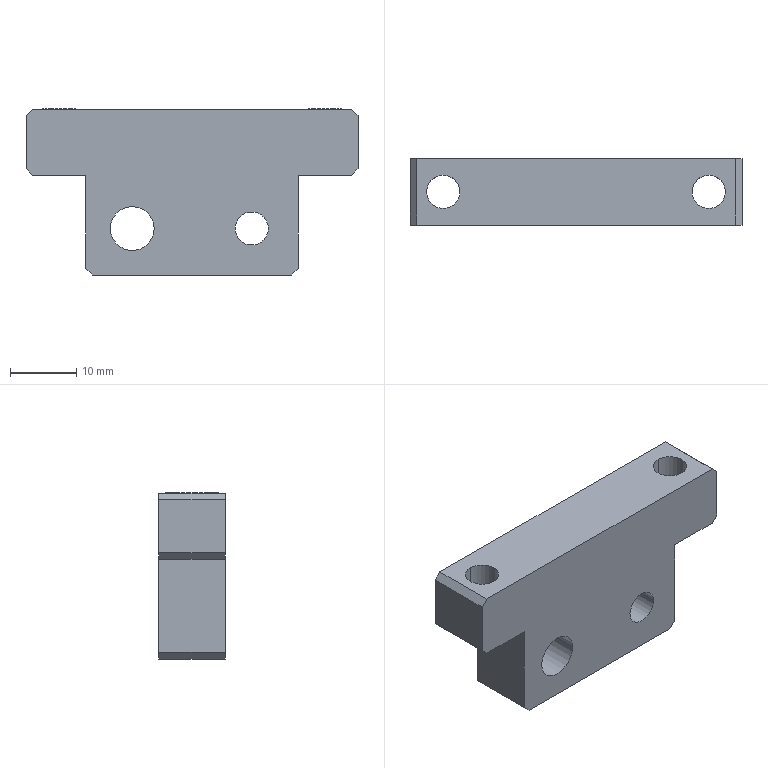Component | SolidWorks | 8TC-A17001-90-08AdjustmentSeat-1 | 1 solid | 24 faces | box 50 x 10 x 25 mm | volume 8839 mm3 | plane 16 | cylinder 8 | commonest cylinder face diameters 5 x6 6.6 x2 | material A3
build123d program:
from build123d import *

# Parameters (mm, degrees)
BOSS_EXTRUDE1_DEPTH                        = 5
THREADED_HOLE_DRILL_FOR_M6_THREADED_HOLE_D = 5
M6_TAPPED_HOLE1_D                          = 5
M6_CLEARANCE_HOLE_1_D                      = 6.6
CHAMFER1_SIZE                              = 1


with BuildPart() as part:
    # Sketch1 → Boss-Extrude1 (new, symmetric)
    with BuildSketch(Plane.XY):
        Polygon((-25, 10), (-16, 10), (-16, 25), (16, 25), (16, 10), (25, 10), (25, 0), (-25, 0), align=None)
    extrude(amount=BOSS_EXTRUDE1_DEPTH, both=True)

    # Threaded Hole Drill for M6 Threaded Hole (through all)
    with Locations(Plane(origin=(0, 10, 0), x_dir=(1, 0, 0), z_dir=(0, 1, 0))):
        with Locations((-20, 0), (20, 0)):
            Hole(THREADED_HOLE_DRILL_FOR_M6_THREADED_HOLE_D / 2)

    # M6 Tapped Hole1 (through all)
    with Locations(Plane.XY.offset(5)):
        with Locations((9, 18)):
            Hole(M6_TAPPED_HOLE1_D / 2)

    # M6 Clearance Hole 1 (through all)
    with Locations(Plane.XY.offset(5)):
        with Locations((-9, 18)):
            Hole(M6_CLEARANCE_HOLE_1_D / 2)

    # Chamfer1
    chamfer1_edges = [part.edges().sort_by_distance(p)[0] for p in [
        (-25, 10, 0),
        (-16, 25, 0),
        (16, 25, 0),
        (25, 10, 0),
        (25, 0, 0),
        (-25, 0, 0),
    ]]
    chamfer(chamfer1_edges, length=CHAMFER1_SIZE)


solid = part.part

# Placed as in the assembly
solid = solid.moved(Location((0, 100, 0), (-90, 0, 0)))
STEP:
#1=COLOUR_RGB('',0.7922,0.8196,0.9333);
#2=FILL_AREA_STYLE_COLOUR('',#1);
#3=FILL_AREA_STYLE('',(#2));
#4=SURFACE_STYLE_FILL_AREA(#3);
#5=SURFACE_SIDE_STYLE('',(#4));
#6=SURFACE_STYLE_USAGE(.BOTH.,#5);
#7=PRESENTATION_STYLE_ASSIGNMENT((#6));
#8=CARTESIAN_POINT('',(-0.4843,3.74,-0.7087));
#9=VERTEX_POINT('',#8);
#10=CARTESIAN_POINT('',(-0.2244,3.74,-0.7087));
#11=VERTEX_POINT('',#10);
#12=CARTESIAN_POINT('',(-0.3543,3.74,-0.7087));
#13=DIRECTION('',(0.,1.,-0.));
#14=DIRECTION('',(1.,0.,0.));
#15=AXIS2_PLACEMENT_3D('',#12,#13,#14);
#16=CIRCLE('',#15,0.1299);
#17=EDGE_CURVE('',#9,#11,#16,.T.);
#18=ORIENTED_EDGE('',*,*,#17,.F.);
#19=CARTESIAN_POINT('',(-0.4843,4.134,-0.7087));
#20=VERTEX_POINT('',#19);
#21=CARTESIAN_POINT('',(-0.4843,4.134,-0.7087));
#22=DIRECTION('',(0.,1.,-0.));
#23=VECTOR('',#22,39.37);
#24=LINE('',#21,#23);
#25=EDGE_CURVE('',#9,#20,#24,.T.);
#26=ORIENTED_EDGE('',*,*,#25,.T.);
#27=CARTESIAN_POINT('',(-0.2244,4.134,-0.7087));
#28=VERTEX_POINT('',#27);
#29=CARTESIAN_POINT('',(-0.3543,4.134,-0.7087));
#30=DIRECTION('',(0.,1.,-0.));
#31=DIRECTION('',(1.,0.,0.));
#32=AXIS2_PLACEMENT_3D('',#29,#30,#31);
#33=CIRCLE('',#32,0.1299);
#34=EDGE_CURVE('',#20,#28,#33,.T.);
#35=ORIENTED_EDGE('',*,*,#34,.T.);
#36=CARTESIAN_POINT('',(-0.2244,4.134,-0.7087));
#37=DIRECTION('',(0.,1.,-0.));
#38=VECTOR('',#37,39.37);
#39=LINE('',#36,#38);
#40=EDGE_CURVE('',#11,#28,#39,.T.);
#41=ORIENTED_EDGE('',*,*,#40,.F.);
#42=EDGE_LOOP('',(#18,#26,#35,#41));
#43=FACE_OUTER_BOUND('',#42,.T.);
#44=CARTESIAN_POINT('',(-0.3543,4.134,-0.7087));
#45=DIRECTION('',(0.,1.,-0.));
#46=DIRECTION('',(1.,0.,0.));
#47=AXIS2_PLACEMENT_3D('',#44,#45,#46);
#48=CYLINDRICAL_SURFACE('',#47,0.1299);
#49=ADVANCED_FACE('',(#43),#48,.F.);
#50=CARTESIAN_POINT('',(0.2559,3.74,-0.7087));
#51=VERTEX_POINT('',#50);
#52=CARTESIAN_POINT('',(0.4528,3.74,-0.7087));
#53=VERTEX_POINT('',#52);
#54=CARTESIAN_POINT('',(0.3543,3.74,-0.7087));
#55=DIRECTION('',(0.,1.,-0.));
#56=DIRECTION('',(1.,0.,0.));
#57=AXIS2_PLACEMENT_3D('',#54,#55,#56);
#58=CIRCLE('',#57,0.09843);
#59=EDGE_CURVE('',#51,#53,#58,.T.);
#60=ORIENTED_EDGE('',*,*,#59,.F.);
#61=CARTESIAN_POINT('',(0.2559,4.134,-0.7087));
#62=VERTEX_POINT('',#61);
#63=CARTESIAN_POINT('',(0.2559,4.134,-0.7087));
#64=DIRECTION('',(0.,1.,-0.));
#65=VECTOR('',#64,39.37);
#66=LINE('',#63,#65);
#67=EDGE_CURVE('',#51,#62,#66,.T.);
#68=ORIENTED_EDGE('',*,*,#67,.T.);
#69=CARTESIAN_POINT('',(0.4528,4.134,-0.7087));
#70=VERTEX_POINT('',#69);
#71=CARTESIAN_POINT('',(0.3543,4.134,-0.7087));
#72=DIRECTION('',(0.,1.,-0.));
#73=DIRECTION('',(1.,0.,0.));
#74=AXIS2_PLACEMENT_3D('',#71,#72,#73);
#75=CIRCLE('',#74,0.09843);
#76=EDGE_CURVE('',#62,#70,#75,.T.);
#77=ORIENTED_EDGE('',*,*,#76,.T.);
#78=CARTESIAN_POINT('',(0.4528,4.134,-0.7087));
#79=DIRECTION('',(0.,1.,-0.));
#80=VECTOR('',#79,39.37);
#81=LINE('',#78,#80);
#82=EDGE_CURVE('',#53,#70,#81,.T.);
#83=ORIENTED_EDGE('',*,*,#82,.F.);
#84=EDGE_LOOP('',(#60,#68,#77,#83));
#85=FACE_OUTER_BOUND('',#84,.T.);
#86=CARTESIAN_POINT('',(0.3543,4.134,-0.7087));
#87=DIRECTION('',(0.,1.,-0.));
#88=DIRECTION('',(1.,0.,0.));
#89=AXIS2_PLACEMENT_3D('',#86,#87,#88);
#90=CYLINDRICAL_SURFACE('',#89,0.09843);
#91=ADVANCED_FACE('',(#85),#90,.F.);
#92=CARTESIAN_POINT('',(-0.7874,3.839,0.));
#93=VERTEX_POINT('',#92);
#94=CARTESIAN_POINT('',(-0.7874,4.035,0.));
#95=VERTEX_POINT('',#94);
#96=CARTESIAN_POINT('',(-0.7874,3.937,0.));
#97=DIRECTION('',(0.,0.,-1.));
#98=DIRECTION('',(0.,1.,0.));
#99=AXIS2_PLACEMENT_3D('',#96,#97,#98);
#100=CIRCLE('',#99,0.09843);
#101=EDGE_CURVE('',#93,#95,#100,.T.);
#102=ORIENTED_EDGE('',*,*,#101,.F.);
#103=CARTESIAN_POINT('',(-0.7874,3.839,-0.3937));
#104=VERTEX_POINT('',#103);
#105=CARTESIAN_POINT('',(-0.7874,3.839,-0.3937));
#106=DIRECTION('',(0.,0.,-1.));
#107=VECTOR('',#106,39.37);
#108=LINE('',#105,#107);
#109=EDGE_CURVE('',#93,#104,#108,.T.);
#110=ORIENTED_EDGE('',*,*,#109,.T.);
#111=CARTESIAN_POINT('',(-0.7874,4.035,-0.3937));
#112=VERTEX_POINT('',#111);
#113=CARTESIAN_POINT('',(-0.7874,3.937,-0.3937));
#114=DIRECTION('',(0.,0.,-1.));
#115=DIRECTION('',(0.,1.,0.));
#116=AXIS2_PLACEMENT_3D('',#113,#114,#115);
#117=CIRCLE('',#116,0.09843);
#118=EDGE_CURVE('',#104,#112,#117,.T.);
#119=ORIENTED_EDGE('',*,*,#118,.T.);
#120=CARTESIAN_POINT('',(-0.7874,4.035,-0.3937));
#121=DIRECTION('',(0.,0.,-1.));
#122=VECTOR('',#121,39.37);
#123=LINE('',#120,#122);
#124=EDGE_CURVE('',#95,#112,#123,.T.);
#125=ORIENTED_EDGE('',*,*,#124,.F.);
#126=EDGE_LOOP('',(#102,#110,#119,#125));
#127=FACE_OUTER_BOUND('',#126,.T.);
#128=CARTESIAN_POINT('',(-0.7874,3.937,-0.3937));
#129=DIRECTION('',(0.,0.,-1.));
#130=DIRECTION('',(0.,1.,0.));
#131=AXIS2_PLACEMENT_3D('',#128,#129,#130);
#132=CYLINDRICAL_SURFACE('',#131,0.09843);
#133=ADVANCED_FACE('',(#127),#132,.F.);
#134=CARTESIAN_POINT('',(0.7874,3.839,0.));
#135=VERTEX_POINT('',#134);
#136=CARTESIAN_POINT('',(0.7874,4.035,0.));
#137=VERTEX_POINT('',#136);
#138=CARTESIAN_POINT('',(0.7874,3.937,0.));
#139=DIRECTION('',(0.,0.,-1.));
#140=DIRECTION('',(0.,1.,0.));
#141=AXIS2_PLACEMENT_3D('',#138,#139,#140);
#142=CIRCLE('',#141,0.09843);
#143=EDGE_CURVE('',#135,#137,#142,.T.);
#144=ORIENTED_EDGE('',*,*,#143,.F.);
#145=CARTESIAN_POINT('',(0.7874,3.839,-0.3937));
#146=VERTEX_POINT('',#145);
#147=CARTESIAN_POINT('',(0.7874,3.839,-0.3937));
#148=DIRECTION('',(0.,0.,-1.));
#149=VECTOR('',#148,39.37);
#150=LINE('',#147,#149);
#151=EDGE_CURVE('',#135,#146,#150,.T.);
#152=ORIENTED_EDGE('',*,*,#151,.T.);
#153=CARTESIAN_POINT('',(0.7874,4.035,-0.3937));
#154=VERTEX_POINT('',#153);
#155=CARTESIAN_POINT('',(0.7874,3.937,-0.3937));
#156=DIRECTION('',(0.,0.,-1.));
#157=DIRECTION('',(0.,1.,0.));
#158=AXIS2_PLACEMENT_3D('',#155,#156,#157);
#159=CIRCLE('',#158,0.09843);
#160=EDGE_CURVE('',#146,#154,#159,.T.);
#161=ORIENTED_EDGE('',*,*,#160,.T.);
#162=CARTESIAN_POINT('',(0.7874,4.035,-0.3937));
#163=DIRECTION('',(0.,0.,-1.));
#164=VECTOR('',#163,39.37);
#165=LINE('',#162,#164);
#166=EDGE_CURVE('',#137,#154,#165,.T.);
#167=ORIENTED_EDGE('',*,*,#166,.F.);
#168=EDGE_LOOP('',(#144,#152,#161,#167));
#169=FACE_OUTER_BOUND('',#168,.T.);
#170=CARTESIAN_POINT('',(0.7874,3.937,-0.3937));
#171=DIRECTION('',(0.,0.,-1.));
#172=DIRECTION('',(0.,1.,0.));
#173=AXIS2_PLACEMENT_3D('',#170,#171,#172);
#174=CYLINDRICAL_SURFACE('',#173,0.09843);
#175=ADVANCED_FACE('',(#169),#174,.F.);
#176=CARTESIAN_POINT('',(-0.9843,4.134,-0.3543));
#177=VERTEX_POINT('',#176);
#178=CARTESIAN_POINT('',(-0.9843,4.134,-0.03937));
#179=VERTEX_POINT('',#178);
#180=CARTESIAN_POINT('',(-0.9843,4.134,-0.3937));
#181=DIRECTION('',(-0.,0.,1.));
#182=VECTOR('',#181,39.37);
#183=LINE('',#180,#182);
#184=EDGE_CURVE('',#177,#179,#183,.T.);
#185=ORIENTED_EDGE('',*,*,#184,.F.);
#186=CARTESIAN_POINT('',(-0.9843,3.74,-0.3543));
#187=VERTEX_POINT('',#186);
#188=CARTESIAN_POINT('',(-0.9843,4.134,-0.3543));
#189=DIRECTION('',(-0.,-1.,0.));
#190=VECTOR('',#189,39.37);
#191=LINE('',#188,#190);
#192=EDGE_CURVE('',#177,#187,#191,.T.);
#193=ORIENTED_EDGE('',*,*,#192,.T.);
#194=CARTESIAN_POINT('',(-0.9843,3.74,-0.03937));
#195=VERTEX_POINT('',#194);
#196=CARTESIAN_POINT('',(-0.9843,3.74,-0.3937));
#197=DIRECTION('',(-0.,0.,1.));
#198=VECTOR('',#197,39.37);
#199=LINE('',#196,#198);
#200=EDGE_CURVE('',#187,#195,#199,.T.);
#201=ORIENTED_EDGE('',*,*,#200,.T.);
#202=CARTESIAN_POINT('',(-0.9843,4.134,-0.03937));
#203=DIRECTION('',(0.,1.,-0.));
#204=VECTOR('',#203,39.37);
#205=LINE('',#202,#204);
#206=EDGE_CURVE('',#195,#179,#205,.T.);
#207=ORIENTED_EDGE('',*,*,#206,.T.);
#208=EDGE_LOOP('',(#185,#193,#201,#207));
#209=FACE_OUTER_BOUND('',#208,.T.);
#210=CARTESIAN_POINT('',(-0.9843,4.134,-0.3937));
#211=DIRECTION('',(1.,-0.,0.));
#212=DIRECTION('',(-0.,-1.,0.));
#213=AXIS2_PLACEMENT_3D('',#210,#211,#212);
#214=PLANE('',#213);
#215=ADVANCED_FACE('',(#209),#214,.F.);
#216=CARTESIAN_POINT('',(-0.7874,3.937,0.));
#217=DIRECTION('',(0.,0.,-1.));
#218=DIRECTION('',(0.,1.,0.));
#219=AXIS2_PLACEMENT_3D('',#216,#217,#218);
#220=CIRCLE('',#219,0.09843);
#221=EDGE_CURVE('',#95,#93,#220,.T.);
#222=ORIENTED_EDGE('',*,*,#221,.T.);
#223=ORIENTED_EDGE('',*,*,#101,.T.);
#224=EDGE_LOOP('',(#222,#223));
#225=FACE_BOUND('',#224,.T.);
#226=CARTESIAN_POINT('',(0.7874,3.937,0.));
#227=DIRECTION('',(0.,0.,-1.));
#228=DIRECTION('',(0.,1.,0.));
#229=AXIS2_PLACEMENT_3D('',#226,#227,#228);
#230=CIRCLE('',#229,0.09843);
#231=EDGE_CURVE('',#137,#135,#230,.T.);
#232=ORIENTED_EDGE('',*,*,#231,.T.);
#233=ORIENTED_EDGE('',*,*,#143,.T.);
#234=EDGE_LOOP('',(#232,#233));
#235=FACE_BOUND('',#234,.T.);
#236=CARTESIAN_POINT('',(-0.9449,3.74,-0.));
#237=VERTEX_POINT('',#236);
#238=CARTESIAN_POINT('',(0.9449,3.74,0.));
#239=VERTEX_POINT('',#238);
#240=CARTESIAN_POINT('',(0.9843,3.74,0.));
#241=DIRECTION('',(1.,0.,0.));
#242=VECTOR('',#241,39.37);
#243=LINE('',#240,#242);
#244=EDGE_CURVE('',#237,#239,#243,.T.);
#245=ORIENTED_EDGE('',*,*,#244,.T.);
#246=CARTESIAN_POINT('',(0.9449,4.134,0.));
#247=VERTEX_POINT('',#246);
#248=CARTESIAN_POINT('',(0.9449,4.134,0.));
#249=DIRECTION('',(0.,1.,-0.));
#250=VECTOR('',#249,39.37);
#251=LINE('',#248,#250);
#252=EDGE_CURVE('',#239,#247,#251,.T.);
#253=ORIENTED_EDGE('',*,*,#252,.T.);
#254=CARTESIAN_POINT('',(-0.9449,4.134,-0.));
#255=VERTEX_POINT('',#254);
#256=CARTESIAN_POINT('',(0.9843,4.134,0.));
#257=DIRECTION('',(1.,0.,0.));
#258=VECTOR('',#257,39.37);
#259=LINE('',#256,#258);
#260=EDGE_CURVE('',#255,#247,#259,.T.);
#261=ORIENTED_EDGE('',*,*,#260,.F.);
#262=CARTESIAN_POINT('',(-0.9449,4.134,-0.));
#263=DIRECTION('',(-0.,-1.,0.));
#264=VECTOR('',#263,39.37);
#265=LINE('',#262,#264);
#266=EDGE_CURVE('',#255,#237,#265,.T.);
#267=ORIENTED_EDGE('',*,*,#266,.T.);
#268=EDGE_LOOP('',(#245,#253,#261,#267));
#269=FACE_OUTER_BOUND('',#268,.T.);
#270=CARTESIAN_POINT('',(0.9843,4.134,0.));
#271=DIRECTION('',(0.,-0.,-1.));
#272=DIRECTION('',(0.,1.,-0.));
#273=AXIS2_PLACEMENT_3D('',#270,#271,#272);
#274=PLANE('',#273);
#275=ADVANCED_FACE('',(#225,#235,#269),#274,.F.);
#276=CARTESIAN_POINT('',(0.9843,3.74,-0.03937));
#277=VERTEX_POINT('',#276);
#278=CARTESIAN_POINT('',(0.9843,3.74,-0.3543));
#279=VERTEX_POINT('',#278);
#280=CARTESIAN_POINT('',(0.9843,3.74,-0.3937));
#281=DIRECTION('',(0.,0.,-1.));
#282=VECTOR('',#281,39.37);
#283=LINE('',#280,#282);
#284=EDGE_CURVE('',#277,#279,#283,.T.);
#285=ORIENTED_EDGE('',*,*,#284,.T.);
#286=CARTESIAN_POINT('',(0.9843,4.134,-0.3543));
#287=VERTEX_POINT('',#286);
#288=CARTESIAN_POINT('',(0.9843,4.134,-0.3543));
#289=DIRECTION('',(0.,1.,-0.));
#290=VECTOR('',#289,39.37);
#291=LINE('',#288,#290);
#292=EDGE_CURVE('',#279,#287,#291,.T.);
#293=ORIENTED_EDGE('',*,*,#292,.T.);
#294=CARTESIAN_POINT('',(0.9843,4.134,-0.03937));
#295=VERTEX_POINT('',#294);
#296=CARTESIAN_POINT('',(0.9843,4.134,-0.3937));
#297=DIRECTION('',(0.,0.,-1.));
#298=VECTOR('',#297,39.37);
#299=LINE('',#296,#298);
#300=EDGE_CURVE('',#295,#287,#299,.T.);
#301=ORIENTED_EDGE('',*,*,#300,.F.);
#302=CARTESIAN_POINT('',(0.9843,4.134,-0.03937));
#303=DIRECTION('',(-0.,-1.,0.));
#304=VECTOR('',#303,39.37);
#305=LINE('',#302,#304);
#306=EDGE_CURVE('',#295,#277,#305,.T.);
#307=ORIENTED_EDGE('',*,*,#306,.T.);
#308=EDGE_LOOP('',(#285,#293,#301,#307));
#309=FACE_OUTER_BOUND('',#308,.T.);
#310=CARTESIAN_POINT('',(0.9843,4.134,-0.3937));
#311=DIRECTION('',(-1.,0.,-0.));
#312=DIRECTION('',(0.,1.,-0.));
#313=AXIS2_PLACEMENT_3D('',#310,#311,#312);
#314=PLANE('',#313);
#315=ADVANCED_FACE('',(#309),#314,.F.);
#316=CARTESIAN_POINT('',(0.7874,3.937,-0.3937));
#317=DIRECTION('',(0.,0.,-1.));
#318=DIRECTION('',(0.,1.,0.));
#319=AXIS2_PLACEMENT_3D('',#316,#317,#318);
#320=CIRCLE('',#319,0.09843);
#321=EDGE_CURVE('',#154,#146,#320,.T.);
#322=ORIENTED_EDGE('',*,*,#321,.F.);
#323=ORIENTED_EDGE('',*,*,#160,.F.);
#324=EDGE_LOOP('',(#322,#323));
#325=FACE_BOUND('',#324,.T.);
#326=CARTESIAN_POINT('',(0.9449,4.134,-0.3937));
#327=VERTEX_POINT('',#326);
#328=CARTESIAN_POINT('',(0.6299,4.134,-0.3937));
#329=VERTEX_POINT('',#328);
#330=CARTESIAN_POINT('',(0.9843,4.134,-0.3937));
#331=DIRECTION('',(-1.,-0.,0.));
#332=VECTOR('',#331,39.37);
#333=LINE('',#330,#332);
#334=EDGE_CURVE('',#327,#329,#333,.T.);
#335=ORIENTED_EDGE('',*,*,#334,.F.);
#336=CARTESIAN_POINT('',(0.9449,3.74,-0.3937));
#337=VERTEX_POINT('',#336);
#338=CARTESIAN_POINT('',(0.9449,4.134,-0.3937));
#339=DIRECTION('',(-0.,-1.,0.));
#340=VECTOR('',#339,39.37);
#341=LINE('',#338,#340);
#342=EDGE_CURVE('',#327,#337,#341,.T.);
#343=ORIENTED_EDGE('',*,*,#342,.T.);
#344=CARTESIAN_POINT('',(0.6299,3.74,-0.3937));
#345=VERTEX_POINT('',#344);
#346=CARTESIAN_POINT('',(0.9843,3.74,-0.3937));
#347=DIRECTION('',(-1.,-0.,0.));
#348=VECTOR('',#347,39.37);
#349=LINE('',#346,#348);
#350=EDGE_CURVE('',#337,#345,#349,.T.);
#351=ORIENTED_EDGE('',*,*,#350,.T.);
#352=CARTESIAN_POINT('',(0.6299,4.134,-0.3937));
#353=DIRECTION('',(-0.,-1.,0.));
#354=VECTOR('',#353,39.37);
#355=LINE('',#352,#354);
#356=EDGE_CURVE('',#329,#345,#355,.T.);
#357=ORIENTED_EDGE('',*,*,#356,.F.);
#358=EDGE_LOOP('',(#335,#343,#351,#357));
#359=FACE_OUTER_BOUND('',#358,.T.);
#360=CARTESIAN_POINT('',(0.9843,4.134,-0.3937));
#361=DIRECTION('',(0.,0.,1.));
#362=DIRECTION('',(1.,0.,-0.));
#363=AXIS2_PLACEMENT_3D('',#360,#361,#362);
#364=PLANE('',#363);
#365=ADVANCED_FACE('',(#325,#359),#364,.F.);
#366=CARTESIAN_POINT('',(0.6299,3.74,-0.9449));
#367=VERTEX_POINT('',#366);
#368=CARTESIAN_POINT('',(0.6299,3.74,-0.3937));
#369=DIRECTION('',(0.,0.,-1.));
#370=VECTOR('',#369,39.37);
#371=LINE('',#368,#370);
#372=EDGE_CURVE('',#345,#367,#371,.T.);
#373=ORIENTED_EDGE('',*,*,#372,.T.);
#374=CARTESIAN_POINT('',(0.6299,4.134,-0.9449));
#375=VERTEX_POINT('',#374);
#376=CARTESIAN_POINT('',(0.6299,4.134,-0.9449));
#377=DIRECTION('',(0.,1.,-0.));
#378=VECTOR('',#377,39.37);
#379=LINE('',#376,#378);
#380=EDGE_CURVE('',#367,#375,#379,.T.);
#381=ORIENTED_EDGE('',*,*,#380,.T.);
#382=CARTESIAN_POINT('',(0.6299,4.134,-0.3937));
#383=DIRECTION('',(0.,0.,-1.));
#384=VECTOR('',#383,39.37);
#385=LINE('',#382,#384);
#386=EDGE_CURVE('',#329,#375,#385,.T.);
#387=ORIENTED_EDGE('',*,*,#386,.F.);
#388=ORIENTED_EDGE('',*,*,#356,.T.);
#389=EDGE_LOOP('',(#373,#381,#387,#388));
#390=FACE_OUTER_BOUND('',#389,.T.);
#391=CARTESIAN_POINT('',(0.6299,4.134,-0.3937));
#392=DIRECTION('',(-1.,0.,-0.));
#393=DIRECTION('',(0.,1.,-0.));
#394=AXIS2_PLACEMENT_3D('',#391,#392,#393);
#395=PLANE('',#394);
#396=ADVANCED_FACE('',(#390),#395,.F.);
#397=CARTESIAN_POINT('',(0.5906,4.134,-0.9843));
#398=VERTEX_POINT('',#397);
#399=CARTESIAN_POINT('',(-0.5906,4.134,-0.9843));
#400=VERTEX_POINT('',#399);
#401=CARTESIAN_POINT('',(0.6299,4.134,-0.9843));
#402=DIRECTION('',(-1.,-0.,-0.));
#403=VECTOR('',#402,39.37);
#404=LINE('',#401,#403);
#405=EDGE_CURVE('',#398,#400,#404,.T.);
#406=ORIENTED_EDGE('',*,*,#405,.F.);
#407=CARTESIAN_POINT('',(0.5906,3.74,-0.9843));
#408=VERTEX_POINT('',#407);
#409=CARTESIAN_POINT('',(0.5906,4.134,-0.9843));
#410=DIRECTION('',(-0.,-1.,0.));
#411=VECTOR('',#410,39.37);
#412=LINE('',#409,#411);
#413=EDGE_CURVE('',#398,#408,#412,.T.);
#414=ORIENTED_EDGE('',*,*,#413,.T.);
#415=CARTESIAN_POINT('',(-0.5906,3.74,-0.9843));
#416=VERTEX_POINT('',#415);
#417=CARTESIAN_POINT('',(0.6299,3.74,-0.9843));
#418=DIRECTION('',(-1.,-0.,-0.));
#419=VECTOR('',#418,39.37);
#420=LINE('',#417,#419);
#421=EDGE_CURVE('',#408,#416,#420,.T.);
#422=ORIENTED_EDGE('',*,*,#421,.T.);
#423=CARTESIAN_POINT('',(-0.5906,4.134,-0.9843));
#424=DIRECTION('',(0.,1.,-0.));
#425=VECTOR('',#424,39.37);
#426=LINE('',#423,#425);
#427=EDGE_CURVE('',#416,#400,#426,.T.);
#428=ORIENTED_EDGE('',*,*,#427,.T.);
#429=EDGE_LOOP('',(#406,#414,#422,#428));
#430=FACE_OUTER_BOUND('',#429,.T.);
#431=CARTESIAN_POINT('',(0.6299,4.134,-0.9843));
#432=DIRECTION('',(-0.,0.,1.));
#433=DIRECTION('',(-0.,-1.,0.));
#434=AXIS2_PLACEMENT_3D('',#431,#432,#433);
#435=PLANE('',#434);
#436=ADVANCED_FACE('',(#430),#435,.F.);
#437=CARTESIAN_POINT('',(-0.6299,4.134,-0.9449));
#438=VERTEX_POINT('',#437);
#439=CARTESIAN_POINT('',(-0.6299,4.134,-0.3937));
#440=VERTEX_POINT('',#439);
#441=CARTESIAN_POINT('',(-0.6299,4.134,-0.3937));
#442=DIRECTION('',(-0.,0.,1.));
#443=VECTOR('',#442,39.37);
#444=LINE('',#441,#443);
#445=EDGE_CURVE('',#438,#440,#444,.T.);
#446=ORIENTED_EDGE('',*,*,#445,.F.);
#447=CARTESIAN_POINT('',(-0.6299,3.74,-0.9449));
#448=VERTEX_POINT('',#447);
#449=CARTESIAN_POINT('',(-0.6299,4.134,-0.9449));
#450=DIRECTION('',(-0.,-1.,0.));
#451=VECTOR('',#450,39.37);
#452=LINE('',#449,#451);
#453=EDGE_CURVE('',#438,#448,#452,.T.);
#454=ORIENTED_EDGE('',*,*,#453,.T.);
#455=CARTESIAN_POINT('',(-0.6299,3.74,-0.3937));
#456=VERTEX_POINT('',#455);
#457=CARTESIAN_POINT('',(-0.6299,3.74,-0.3937));
#458=DIRECTION('',(-0.,0.,1.));
#459=VECTOR('',#458,39.37);
#460=LINE('',#457,#459);
#461=EDGE_CURVE('',#448,#456,#460,.T.);
#462=ORIENTED_EDGE('',*,*,#461,.T.);
#463=CARTESIAN_POINT('',(-0.6299,4.134,-0.3937));
#464=DIRECTION('',(-0.,-1.,0.));
#465=VECTOR('',#464,39.37);
#466=LINE('',#463,#465);
#467=EDGE_CURVE('',#440,#456,#466,.T.);
#468=ORIENTED_EDGE('',*,*,#467,.F.);
#469=EDGE_LOOP('',(#446,#454,#462,#468));
#470=FACE_OUTER_BOUND('',#469,.T.);
#471=CARTESIAN_POINT('',(-0.6299,4.134,-0.3937));
#472=DIRECTION('',(1.,-0.,0.));
#473=DIRECTION('',(-0.,-1.,0.));
#474=AXIS2_PLACEMENT_3D('',#471,#472,#473);
#475=PLANE('',#474);
#476=ADVANCED_FACE('',(#470),#475,.F.);
#477=CARTESIAN_POINT('',(-0.7874,3.937,-0.3937));
#478=DIRECTION('',(0.,0.,-1.));
#479=DIRECTION('',(0.,1.,0.));
#480=AXIS2_PLACEMENT_3D('',#477,#478,#479);
#481=CIRCLE('',#480,0.09843);
#482=EDGE_CURVE('',#112,#104,#481,.T.);
#483=ORIENTED_EDGE('',*,*,#482,.F.);
#484=ORIENTED_EDGE('',*,*,#118,.F.);
#485=EDGE_LOOP('',(#483,#484));
#486=FACE_BOUND('',#485,.T.);
#487=CARTESIAN_POINT('',(-0.9449,3.74,-0.3937));
#488=VERTEX_POINT('',#487);
#489=CARTESIAN_POINT('',(-0.9843,3.74,-0.3937));
#490=DIRECTION('',(-1.,-0.,-0.));
#491=VECTOR('',#490,39.37);
#492=LINE('',#489,#491);
#493=EDGE_CURVE('',#456,#488,#492,.T.);
#494=ORIENTED_EDGE('',*,*,#493,.T.);
#495=CARTESIAN_POINT('',(-0.9449,4.134,-0.3937));
#496=VERTEX_POINT('',#495);
#497=CARTESIAN_POINT('',(-0.9449,4.134,-0.3937));
#498=DIRECTION('',(0.,1.,-0.));
#499=VECTOR('',#498,39.37);
#500=LINE('',#497,#499);
#501=EDGE_CURVE('',#488,#496,#500,.T.);
#502=ORIENTED_EDGE('',*,*,#501,.T.);
#503=CARTESIAN_POINT('',(-0.9843,4.134,-0.3937));
#504=DIRECTION('',(-1.,-0.,-0.));
#505=VECTOR('',#504,39.37);
#506=LINE('',#503,#505);
#507=EDGE_CURVE('',#440,#496,#506,.T.);
#508=ORIENTED_EDGE('',*,*,#507,.F.);
#509=ORIENTED_EDGE('',*,*,#467,.T.);
#510=EDGE_LOOP('',(#494,#502,#508,#509));
#511=FACE_OUTER_BOUND('',#510,.T.);
#512=CARTESIAN_POINT('',(-0.9843,4.134,-0.3937));
#513=DIRECTION('',(-0.,-0.,1.));
#514=DIRECTION('',(1.,0.,0.));
#515=AXIS2_PLACEMENT_3D('',#512,#513,#514);
#516=PLANE('',#515);
#517=ADVANCED_FACE('',(#486,#511),#516,.F.);
#518=CARTESIAN_POINT('',(-0.3543,4.134,-0.7087));
#519=DIRECTION('',(0.,1.,-0.));
#520=DIRECTION('',(1.,0.,0.));
#521=AXIS2_PLACEMENT_3D('',#518,#519,#520);
#522=CIRCLE('',#521,0.1299);
#523=EDGE_CURVE('',#28,#20,#522,.T.);
#524=ORIENTED_EDGE('',*,*,#523,.F.);
#525=ORIENTED_EDGE('',*,*,#34,.F.);
#526=EDGE_LOOP('',(#524,#525));
#527=FACE_BOUND('',#526,.T.);
#528=CARTESIAN_POINT('',(0.3543,4.134,-0.7087));
#529=DIRECTION('',(0.,1.,-0.));
#530=DIRECTION('',(1.,0.,0.));
#531=AXIS2_PLACEMENT_3D('',#528,#529,#530);
#532=CIRCLE('',#531,0.09843);
#533=EDGE_CURVE('',#70,#62,#532,.T.);
#534=ORIENTED_EDGE('',*,*,#533,.F.);
#535=ORIENTED_EDGE('',*,*,#76,.F.);
#536=EDGE_LOOP('',(#534,#535));
#537=FACE_BOUND('',#536,.T.);
#538=ORIENTED_EDGE('',*,*,#507,.T.);
#539=CARTESIAN_POINT('',(-0.9843,4.134,-0.3543));
#540=DIRECTION('',(-0.7071,-0.,0.7071));
#541=VECTOR('',#540,39.37);
#542=LINE('',#539,#541);
#543=EDGE_CURVE('',#496,#177,#542,.T.);
#544=ORIENTED_EDGE('',*,*,#543,.T.);
#545=ORIENTED_EDGE('',*,*,#184,.T.);
#546=CARTESIAN_POINT('',(-0.9449,4.134,-0.));
#547=DIRECTION('',(0.7071,0.,0.7071));
#548=VECTOR('',#547,39.37);
#549=LINE('',#546,#548);
#550=EDGE_CURVE('',#179,#255,#549,.T.);
#551=ORIENTED_EDGE('',*,*,#550,.T.);
#552=ORIENTED_EDGE('',*,*,#260,.T.);
#553=CARTESIAN_POINT('',(0.9843,4.134,-0.03937));
#554=DIRECTION('',(0.7071,0.,-0.7071));
#555=VECTOR('',#554,39.37);
#556=LINE('',#553,#555);
#557=EDGE_CURVE('',#247,#295,#556,.T.);
#558=ORIENTED_EDGE('',*,*,#557,.T.);
#559=ORIENTED_EDGE('',*,*,#300,.T.);
#560=CARTESIAN_POINT('',(0.9449,4.134,-0.3937));
#561=DIRECTION('',(-0.7071,-0.,-0.7071));
#562=VECTOR('',#561,39.37);
#563=LINE('',#560,#562);
#564=EDGE_CURVE('',#287,#327,#563,.T.);
#565=ORIENTED_EDGE('',*,*,#564,.T.);
#566=ORIENTED_EDGE('',*,*,#334,.T.);
#567=ORIENTED_EDGE('',*,*,#386,.T.);
#568=CARTESIAN_POINT('',(0.5906,4.134,-0.9843));
#569=DIRECTION('',(-0.7071,-0.,-0.7071));
#570=VECTOR('',#569,39.37);
#571=LINE('',#568,#570);
#572=EDGE_CURVE('',#375,#398,#571,.T.);
#573=ORIENTED_EDGE('',*,*,#572,.T.);
#574=ORIENTED_EDGE('',*,*,#405,.T.);
#575=CARTESIAN_POINT('',(-0.6299,4.134,-0.9449));
#576=DIRECTION('',(-0.7071,-0.,0.7071));
#577=VECTOR('',#576,39.37);
#578=LINE('',#575,#577);
#579=EDGE_CURVE('',#400,#438,#578,.T.);
#580=ORIENTED_EDGE('',*,*,#579,.T.);
#581=ORIENTED_EDGE('',*,*,#445,.T.);
#582=EDGE_LOOP('',(#538,#544,#545,#551,#552,#558,#559,#565,#566,#567,#573,#574,#580,#581));
#583=FACE_OUTER_BOUND('',#582,.T.);
#584=CARTESIAN_POINT('',(-0.,4.134,-0.));
#585=DIRECTION('',(0.,-1.,0.));
#586=DIRECTION('',(-1.,-0.,-0.));
#587=AXIS2_PLACEMENT_3D('',#584,#585,#586);
#588=PLANE('',#587);
#589=ADVANCED_FACE('',(#527,#537,#583),#588,.F.);
#590=CARTESIAN_POINT('',(-0.3543,3.74,-0.7087));
#591=DIRECTION('',(0.,1.,-0.));
#592=DIRECTION('',(1.,0.,0.));
#593=AXIS2_PLACEMENT_3D('',#590,#591,#592);
#594=CIRCLE('',#593,0.1299);
#595=EDGE_CURVE('',#11,#9,#594,.T.);
#596=ORIENTED_EDGE('',*,*,#595,.T.);
#597=ORIENTED_EDGE('',*,*,#17,.T.);
#598=EDGE_LOOP('',(#596,#597));
#599=FACE_BOUND('',#598,.T.);
#600=CARTESIAN_POINT('',(0.3543,3.74,-0.7087));
#601=DIRECTION('',(0.,1.,-0.));
#602=DIRECTION('',(1.,0.,0.));
#603=AXIS2_PLACEMENT_3D('',#600,#601,#602);
#604=CIRCLE('',#603,0.09843);
#605=EDGE_CURVE('',#53,#51,#604,.T.);
#606=ORIENTED_EDGE('',*,*,#605,.T.);
#607=ORIENTED_EDGE('',*,*,#59,.T.);
#608=EDGE_LOOP('',(#606,#607));
#609=FACE_BOUND('',#608,.T.);
#610=ORIENTED_EDGE('',*,*,#200,.F.);
#611=CARTESIAN_POINT('',(-0.6693,3.74,-0.6693));
#612=DIRECTION('',(0.7071,0.,-0.7071));
#613=VECTOR('',#612,39.37);
#614=LINE('',#611,#613);
#615=EDGE_CURVE('',#187,#488,#614,.T.);
#616=ORIENTED_EDGE('',*,*,#615,.T.);
#617=ORIENTED_EDGE('',*,*,#493,.F.);
#618=ORIENTED_EDGE('',*,*,#461,.F.);
#619=CARTESIAN_POINT('',(-0.7874,3.74,-0.7874));
#620=DIRECTION('',(0.7071,0.,-0.7071));
#621=VECTOR('',#620,39.37);
#622=LINE('',#619,#621);
#623=EDGE_CURVE('',#448,#416,#622,.T.);
#624=ORIENTED_EDGE('',*,*,#623,.T.);
#625=ORIENTED_EDGE('',*,*,#421,.F.);
#626=CARTESIAN_POINT('',(0.7874,3.74,-0.7874));
#627=DIRECTION('',(0.7071,0.,0.7071));
#628=VECTOR('',#627,39.37);
#629=LINE('',#626,#628);
#630=EDGE_CURVE('',#408,#367,#629,.T.);
#631=ORIENTED_EDGE('',*,*,#630,.T.);
#632=ORIENTED_EDGE('',*,*,#372,.F.);
#633=ORIENTED_EDGE('',*,*,#350,.F.);
#634=CARTESIAN_POINT('',(0.6693,3.74,-0.6693));
#635=DIRECTION('',(0.7071,0.,0.7071));
#636=VECTOR('',#635,39.37);
#637=LINE('',#634,#636);
#638=EDGE_CURVE('',#337,#279,#637,.T.);
#639=ORIENTED_EDGE('',*,*,#638,.T.);
#640=ORIENTED_EDGE('',*,*,#284,.F.);
#641=CARTESIAN_POINT('',(0.4724,3.74,0.4724));
#642=DIRECTION('',(-0.7071,-0.,0.7071));
#643=VECTOR('',#642,39.37);
#644=LINE('',#641,#643);
#645=EDGE_CURVE('',#277,#239,#644,.T.);
#646=ORIENTED_EDGE('',*,*,#645,.T.);
#647=ORIENTED_EDGE('',*,*,#244,.F.);
#648=CARTESIAN_POINT('',(-0.4724,3.74,0.4724));
#649=DIRECTION('',(-0.7071,-0.,-0.7071));
#650=VECTOR('',#649,39.37);
#651=LINE('',#648,#650);
#652=EDGE_CURVE('',#237,#195,#651,.T.);
#653=ORIENTED_EDGE('',*,*,#652,.T.);
#654=EDGE_LOOP('',(#610,#616,#617,#618,#624,#625,#631,#632,#633,#639,#640,#646,#647,#653));
#655=FACE_OUTER_BOUND('',#654,.T.);
#656=CARTESIAN_POINT('',(-0.,3.74,-0.));
#657=DIRECTION('',(0.,-1.,0.));
#658=DIRECTION('',(-1.,-0.,-0.));
#659=AXIS2_PLACEMENT_3D('',#656,#657,#658);
#660=PLANE('',#659);
#661=ADVANCED_FACE('',(#599,#609,#655),#660,.T.);
#662=ORIENTED_EDGE('',*,*,#151,.F.);
#663=ORIENTED_EDGE('',*,*,#231,.F.);
#664=ORIENTED_EDGE('',*,*,#166,.T.);
#665=ORIENTED_EDGE('',*,*,#321,.T.);
#666=EDGE_LOOP('',(#662,#663,#664,#665));
#667=FACE_OUTER_BOUND('',#666,.T.);
#668=CARTESIAN_POINT('',(0.7874,3.937,-0.3937));
#669=DIRECTION('',(0.,0.,-1.));
#670=DIRECTION('',(0.,1.,0.));
#671=AXIS2_PLACEMENT_3D('',#668,#669,#670);
#672=CYLINDRICAL_SURFACE('',#671,0.09843);
#673=ADVANCED_FACE('',(#667),#672,.F.);
#674=ORIENTED_EDGE('',*,*,#109,.F.);
#675=ORIENTED_EDGE('',*,*,#221,.F.);
#676=ORIENTED_EDGE('',*,*,#124,.T.);
#677=ORIENTED_EDGE('',*,*,#482,.T.);
#678=EDGE_LOOP('',(#674,#675,#676,#677));
#679=FACE_OUTER_BOUND('',#678,.T.);
#680=CARTESIAN_POINT('',(-0.7874,3.937,-0.3937));
#681=DIRECTION('',(0.,0.,-1.));
#682=DIRECTION('',(0.,1.,0.));
#683=AXIS2_PLACEMENT_3D('',#680,#681,#682);
#684=CYLINDRICAL_SURFACE('',#683,0.09843);
#685=ADVANCED_FACE('',(#679),#684,.F.);
#686=ORIENTED_EDGE('',*,*,#67,.F.);
#687=ORIENTED_EDGE('',*,*,#605,.F.);
#688=ORIENTED_EDGE('',*,*,#82,.T.);
#689=ORIENTED_EDGE('',*,*,#533,.T.);
#690=EDGE_LOOP('',(#686,#687,#688,#689));
#691=FACE_OUTER_BOUND('',#690,.T.);
#692=CARTESIAN_POINT('',(0.3543,4.134,-0.7087));
#693=DIRECTION('',(0.,1.,-0.));
#694=DIRECTION('',(1.,0.,0.));
#695=AXIS2_PLACEMENT_3D('',#692,#693,#694);
#696=CYLINDRICAL_SURFACE('',#695,0.09843);
#697=ADVANCED_FACE('',(#691),#696,.F.);
#698=ORIENTED_EDGE('',*,*,#25,.F.);
#699=ORIENTED_EDGE('',*,*,#595,.F.);
#700=ORIENTED_EDGE('',*,*,#40,.T.);
#701=ORIENTED_EDGE('',*,*,#523,.T.);
#702=EDGE_LOOP('',(#698,#699,#700,#701));
#703=FACE_OUTER_BOUND('',#702,.T.);
#704=CARTESIAN_POINT('',(-0.3543,4.134,-0.7087));
#705=DIRECTION('',(0.,1.,-0.));
#706=DIRECTION('',(1.,0.,0.));
#707=AXIS2_PLACEMENT_3D('',#704,#705,#706);
#708=CYLINDRICAL_SURFACE('',#707,0.1299);
#709=ADVANCED_FACE('',(#703),#708,.F.);
#710=ORIENTED_EDGE('',*,*,#543,.F.);
#711=ORIENTED_EDGE('',*,*,#501,.F.);
#712=ORIENTED_EDGE('',*,*,#615,.F.);
#713=ORIENTED_EDGE('',*,*,#192,.F.);
#714=EDGE_LOOP('',(#710,#711,#712,#713));
#715=FACE_OUTER_BOUND('',#714,.T.);
#716=CARTESIAN_POINT('',(-0.9843,4.134,-0.3543));
#717=DIRECTION('',(0.7071,0.,0.7071));
#718=DIRECTION('',(-0.,-1.,0.));
#719=AXIS2_PLACEMENT_3D('',#716,#717,#718);
#720=PLANE('',#719);
#721=ADVANCED_FACE('',(#715),#720,.F.);
#722=ORIENTED_EDGE('',*,*,#572,.F.);
#723=ORIENTED_EDGE('',*,*,#380,.F.);
#724=ORIENTED_EDGE('',*,*,#630,.F.);
#725=ORIENTED_EDGE('',*,*,#413,.F.);
#726=EDGE_LOOP('',(#722,#723,#724,#725));
#727=FACE_OUTER_BOUND('',#726,.T.);
#728=CARTESIAN_POINT('',(0.5906,4.134,-0.9843));
#729=DIRECTION('',(-0.7071,0.,0.7071));
#730=DIRECTION('',(-0.,-1.,0.));
#731=AXIS2_PLACEMENT_3D('',#728,#729,#730);
#732=PLANE('',#731);
#733=ADVANCED_FACE('',(#727),#732,.F.);
#734=ORIENTED_EDGE('',*,*,#564,.F.);
#735=ORIENTED_EDGE('',*,*,#292,.F.);
#736=ORIENTED_EDGE('',*,*,#638,.F.);
#737=ORIENTED_EDGE('',*,*,#342,.F.);
#738=EDGE_LOOP('',(#734,#735,#736,#737));
#739=FACE_OUTER_BOUND('',#738,.T.);
#740=CARTESIAN_POINT('',(0.9449,4.134,-0.3937));
#741=DIRECTION('',(-0.7071,0.,0.7071));
#742=DIRECTION('',(-0.,-1.,0.));
#743=AXIS2_PLACEMENT_3D('',#740,#741,#742);
#744=PLANE('',#743);
#745=ADVANCED_FACE('',(#739),#744,.F.);
#746=ORIENTED_EDGE('',*,*,#557,.F.);
#747=ORIENTED_EDGE('',*,*,#252,.F.);
#748=ORIENTED_EDGE('',*,*,#645,.F.);
#749=ORIENTED_EDGE('',*,*,#306,.F.);
#750=EDGE_LOOP('',(#746,#747,#748,#749));
#751=FACE_OUTER_BOUND('',#750,.T.);
#752=CARTESIAN_POINT('',(0.9843,4.134,-0.03937));
#753=DIRECTION('',(-0.7071,-0.,-0.7071));
#754=DIRECTION('',(-0.,-1.,0.));
#755=AXIS2_PLACEMENT_3D('',#752,#753,#754);
#756=PLANE('',#755);
#757=ADVANCED_FACE('',(#751),#756,.F.);
#758=ORIENTED_EDGE('',*,*,#550,.F.);
#759=ORIENTED_EDGE('',*,*,#206,.F.);
#760=ORIENTED_EDGE('',*,*,#652,.F.);
#761=ORIENTED_EDGE('',*,*,#266,.F.);
#762=EDGE_LOOP('',(#758,#759,#760,#761));
#763=FACE_OUTER_BOUND('',#762,.T.);
#764=CARTESIAN_POINT('',(-0.9449,4.134,-0.));
#765=DIRECTION('',(0.7071,-0.,-0.7071));
#766=DIRECTION('',(-0.,-1.,0.));
#767=AXIS2_PLACEMENT_3D('',#764,#765,#766);
#768=PLANE('',#767);
#769=ADVANCED_FACE('',(#763),#768,.F.);
#770=ORIENTED_EDGE('',*,*,#579,.F.);
#771=ORIENTED_EDGE('',*,*,#427,.F.);
#772=ORIENTED_EDGE('',*,*,#623,.F.);
#773=ORIENTED_EDGE('',*,*,#453,.F.);
#774=EDGE_LOOP('',(#770,#771,#772,#773));
#775=FACE_OUTER_BOUND('',#774,.T.);
#776=CARTESIAN_POINT('',(-0.6299,4.134,-0.9449));
#777=DIRECTION('',(0.7071,0.,0.7071));
#778=DIRECTION('',(-0.,-1.,0.));
#779=AXIS2_PLACEMENT_3D('',#776,#777,#778);
#780=PLANE('',#779);
#781=ADVANCED_FACE('',(#775),#780,.F.);
#782=CLOSED_SHELL('',(#49,#91,#133,#175,#215,#275,#315,#365,#396,#436,#476,#517,#589,#661,#673,#685,#697,#709,#721,#733,#745,#757,#769,#781));
#783=MANIFOLD_SOLID_BREP('',#782);
#784=STYLED_ITEM('',(#7),#783);
#785=(LENGTH_UNIT()NAMED_UNIT(*)SI_UNIT($,.METRE.));
#786=LENGTH_MEASURE_WITH_UNIT(LENGTH_MEASURE(0.0254),#785);
#787=DIMENSIONAL_EXPONENTS(1.,0.,0.,0.,0.,0.,0.);
#788=(CONVERSION_BASED_UNIT('',#786)LENGTH_UNIT()NAMED_UNIT(#787));
#789=UNCERTAINTY_MEASURE_WITH_UNIT(LENGTH_MEASURE(0.00001),#788,'','');
#790=(NAMED_UNIT(*)PLANE_ANGLE_UNIT()SI_UNIT($,.RADIAN.));
#791=(NAMED_UNIT(*)SI_UNIT($,.STERADIAN.)SOLID_ANGLE_UNIT());
#792=(GEOMETRIC_REPRESENTATION_CONTEXT(3)GLOBAL_UNCERTAINTY_ASSIGNED_CONTEXT((#789))GLOBAL_UNIT_ASSIGNED_CONTEXT((#788,#790,#791))REPRESENTATION_CONTEXT('',''));
#793=MECHANICAL_DESIGN_GEOMETRIC_PRESENTATION_REPRESENTATION('',(#784),#792);
#794=PRESENTATION_LAYER_ASSIGNMENT('','',(#784));
#795=CARTESIAN_POINT('',(0.,0.,0.));
#796=DIRECTION('',(0.,0.,1.));
#797=DIRECTION('',(1.,0.,0.));
#798=AXIS2_PLACEMENT_3D('',#795,#796,#797);
#799=(LENGTH_UNIT()NAMED_UNIT(*)SI_UNIT($,.METRE.));
#800=LENGTH_MEASURE_WITH_UNIT(LENGTH_MEASURE(0.0254),#799);
#801=DIMENSIONAL_EXPONENTS(1.,0.,0.,0.,0.,0.,0.);
#802=(CONVERSION_BASED_UNIT('',#800)LENGTH_UNIT()NAMED_UNIT(#801));
#803=UNCERTAINTY_MEASURE_WITH_UNIT(LENGTH_MEASURE(0.00001),#802,'','');
#804=(NAMED_UNIT(*)PLANE_ANGLE_UNIT()SI_UNIT($,.RADIAN.));
#805=(NAMED_UNIT(*)SI_UNIT($,.STERADIAN.)SOLID_ANGLE_UNIT());
#806=(GEOMETRIC_REPRESENTATION_CONTEXT(3)GLOBAL_UNCERTAINTY_ASSIGNED_CONTEXT((#803))GLOBAL_UNIT_ASSIGNED_CONTEXT((#802,#804,#805))REPRESENTATION_CONTEXT('',''));
#807=ADVANCED_BREP_SHAPE_REPRESENTATION('',(#783,#798),#806);